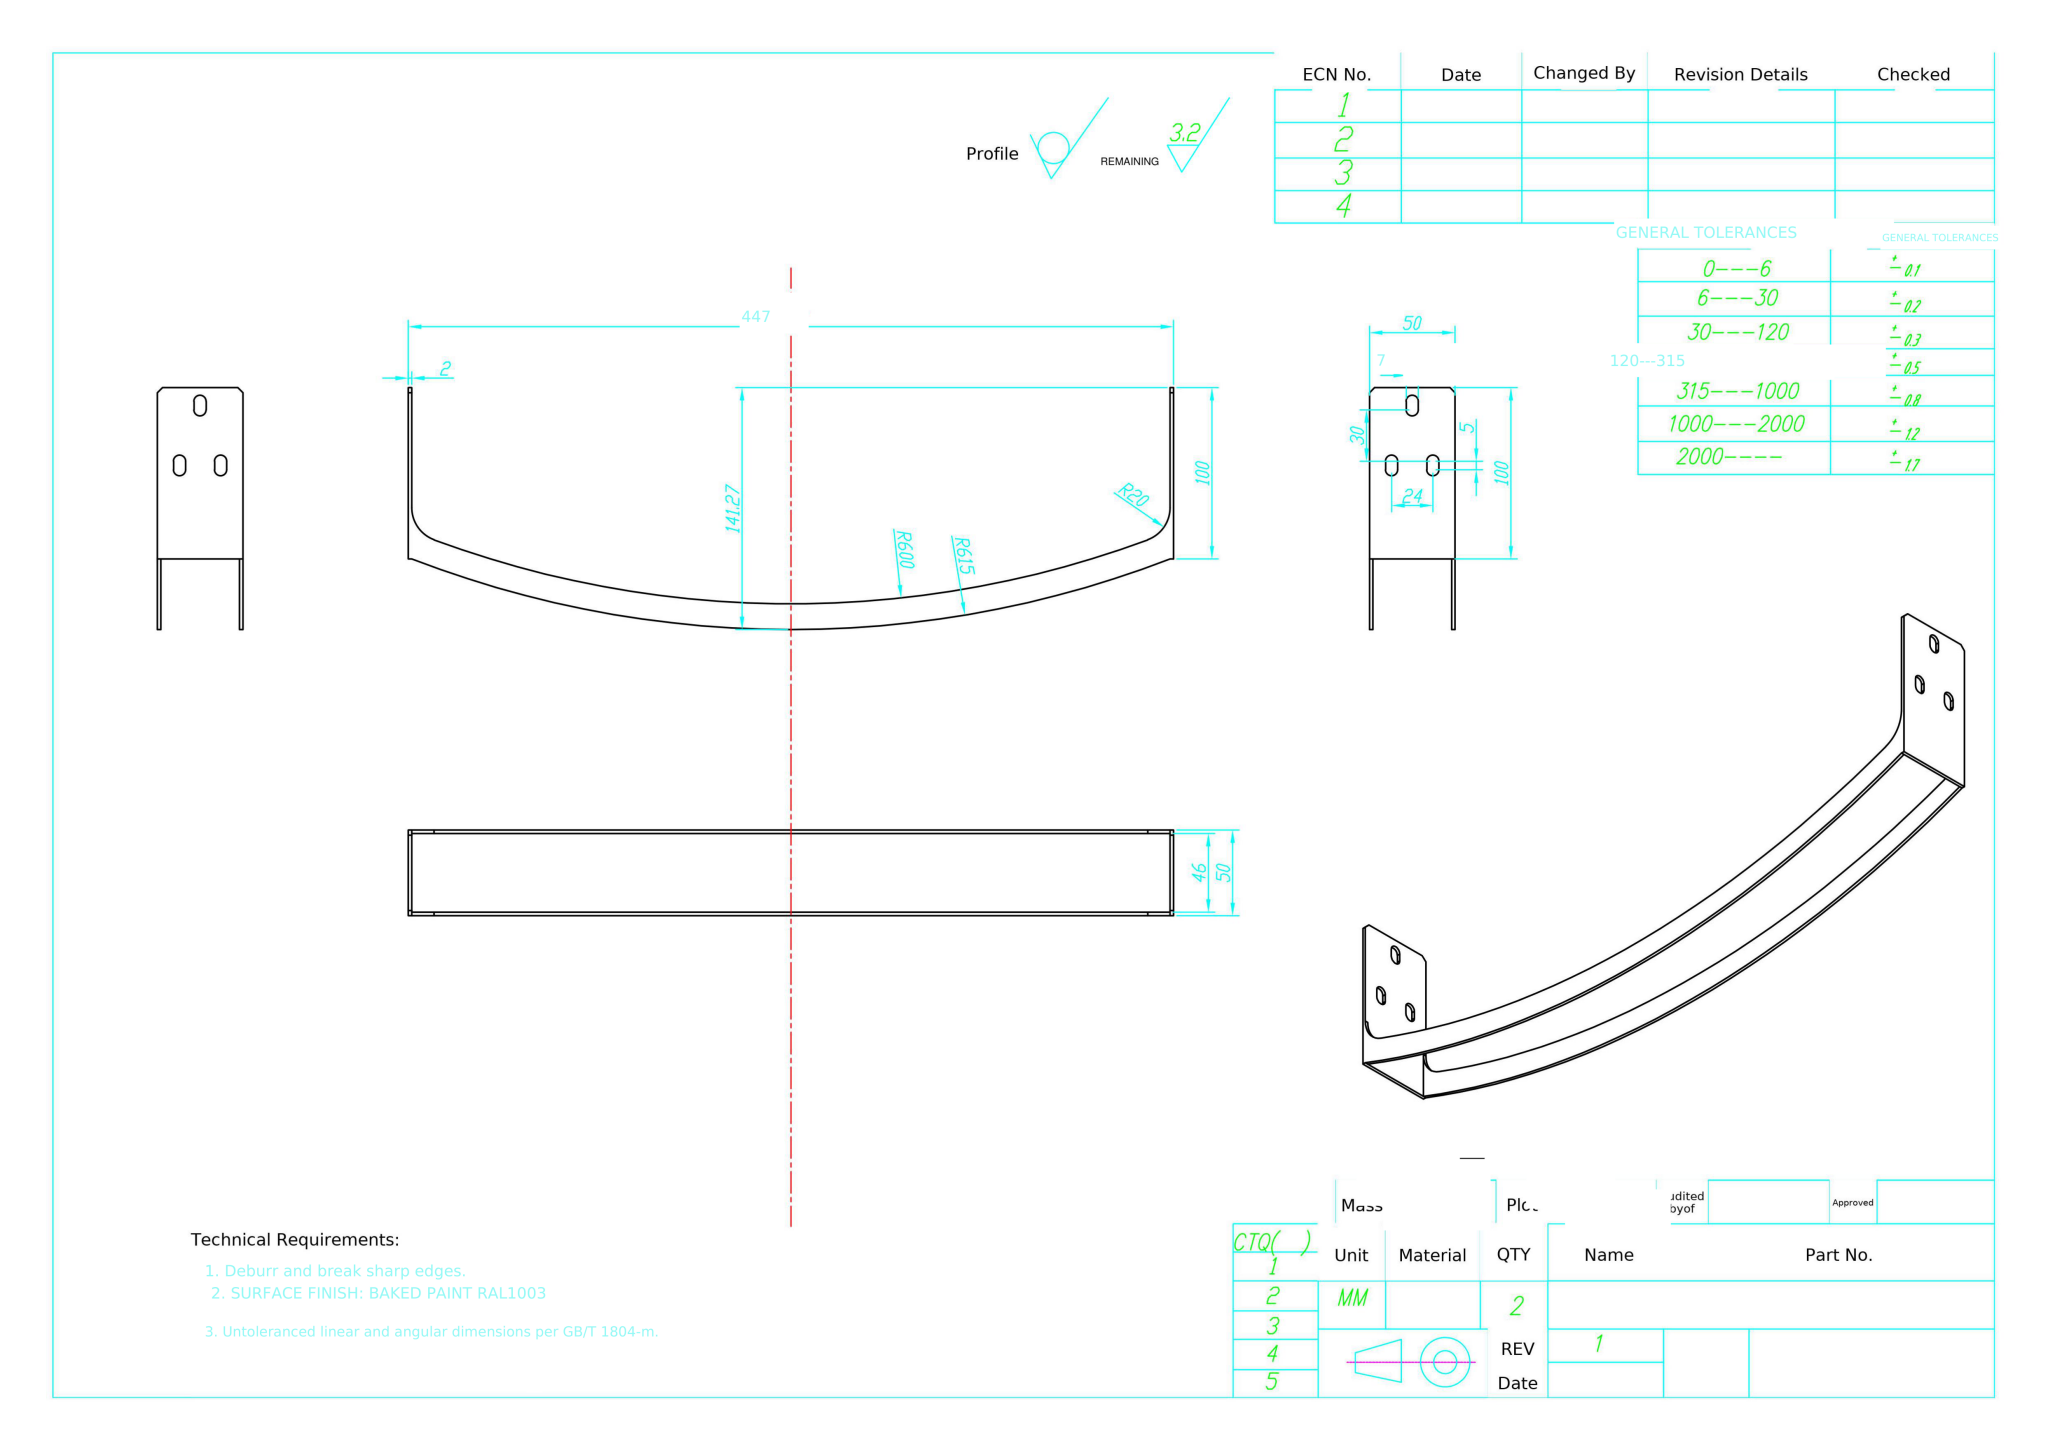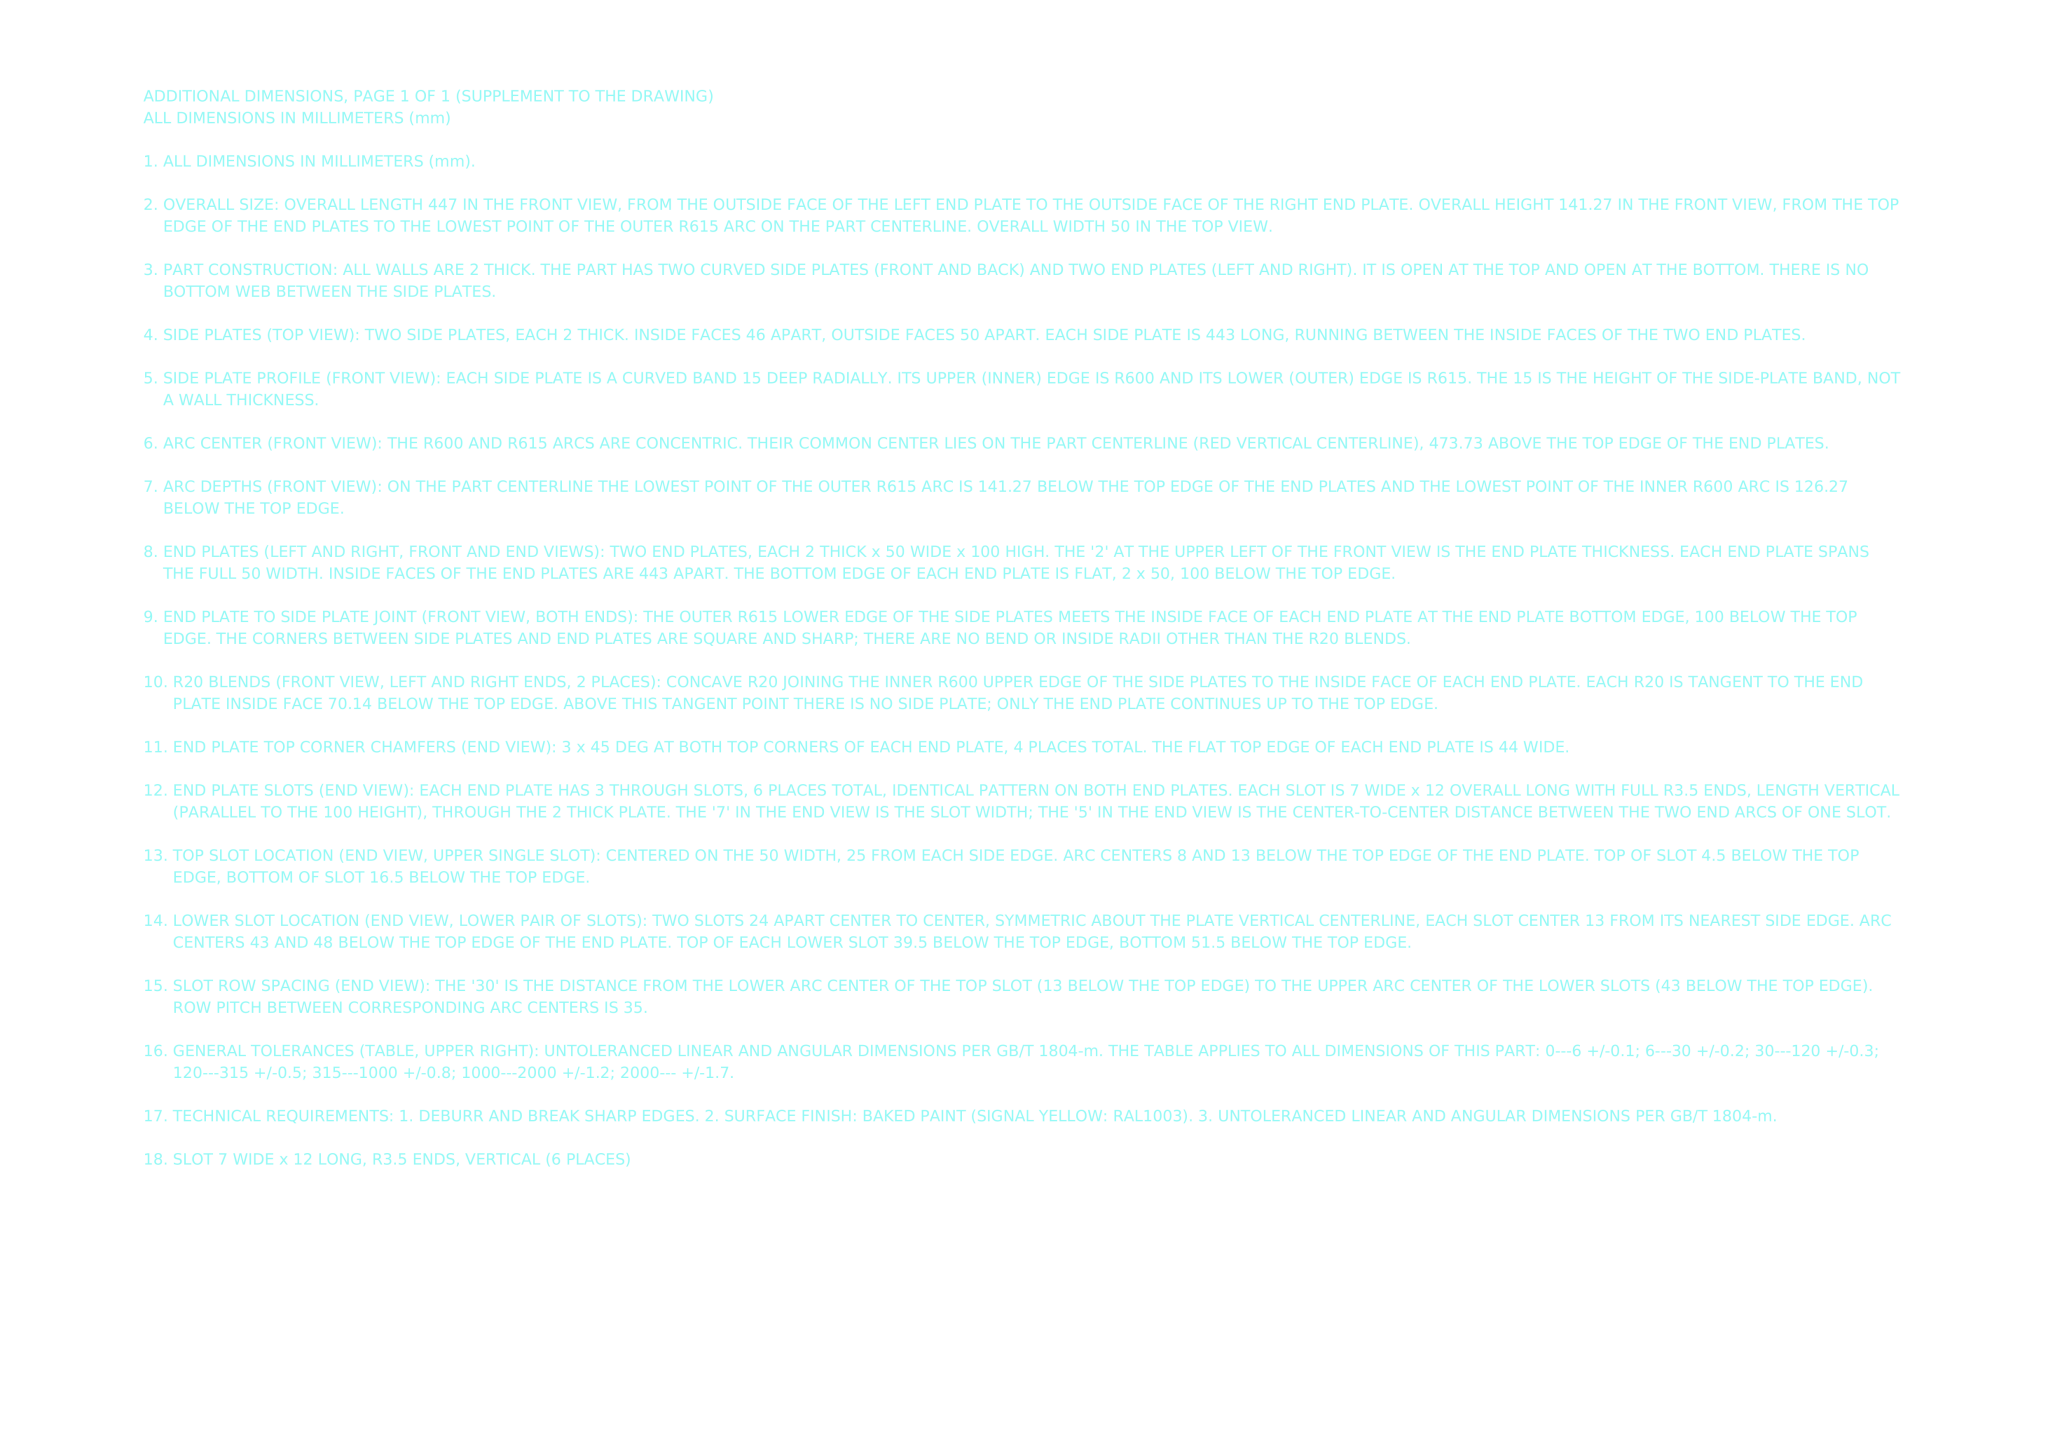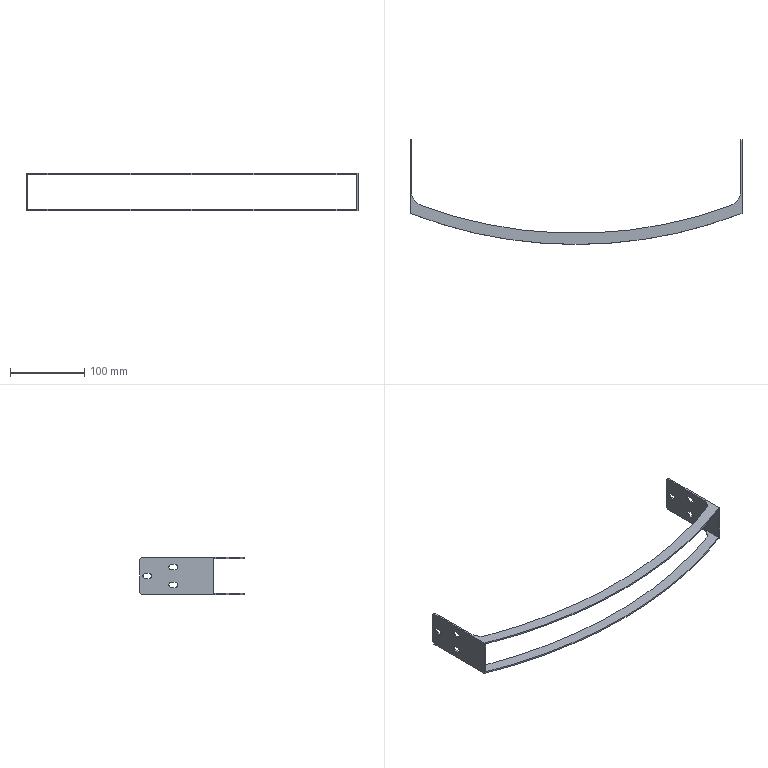Part | NX | mm | 1 solid | 48 faces | box 447 x 141.27 x 50 mm | volume 46565 mm3 | plane 28 | cylinder 20 | commonest cylinder face diameters 7 x12 40 x4 1200 x2 1230 x2